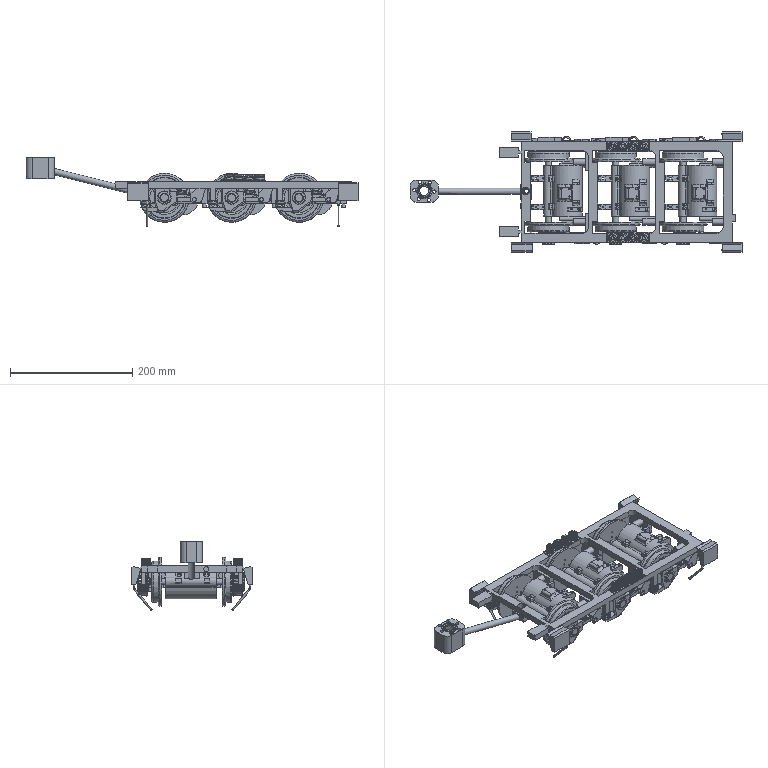Assembly | NX | mm | 34 component files | 77 solids | 1892 faces | box 542.92 x 197.4 x 112.37 mm | volume 1368528 mm3 | plane 1259 | cylinder 414 | spline 106 | sphere 64 | torus 49 | commonest cylinder face diameters 6 x108 2.235 x36 2.354 x36 7.6 x18 4.56 x12 10 x10 20 x10 10.2 x9
Bill of materials:
unnamed part 1 | 6 |  | Compact multi-body bracket/latch-like piece: blocky central body with a raised rounded-rectangle top pad and a circular boss with concentric stepped rings on one face, a curved-bottom wedge-shaped flange projecting to one side, and a slender bar extending the other way to an angled plate tab with a round through-hole.
unnamed part 2 | 1 |  | Rectangular ladder-style open frame: two long side rails joined by end and intermediate cross members, making three open bays. Small blocks and short cylindrical pins hang below, block-shaped end pieces sit at the four corners, thin angled rods extend downward and outward at the ends, and small raised studs run in a row along parts of the rails.
unnamed part 3 | 3 |  | Wheel-and-axle-like body: two identical flanged discs on the ends of a straight cylindrical shaft. Each disc has a larger-diameter flange lip on its inner side, a recessed face, and a ring pattern of small round holes or dimples. The shaft ends stick out a little past the discs.
unnamed part 4 | 3 |  | Large cylindrical body with a smaller parallel tube along one side. Raised saddle/rib features and a square mounting pad with small holes sit on top, and two flat perforated strip tabs stick out sideways. The end face has an off-center through-hole, a lug ring around the side tube bore, and a straight arm extending from that lug.
unnamed part 5 | 20 |  | Helical coil of round-section wire wound closely, about 7–8 turns, with a flat ground-style annular face at the top end and an open bore through the center.
unnamed part 6 | 1 |  | Two blocks joined by a long straight cylindrical rod: a larger rounded-square block with a central bore, an encircling ring of small spherical bumps, and four corner holes, and a small rectangular block at the far end with its own small bore ringed by small bumps. The rod meets the large block on its side face and runs at an angle.
Mates:
1. touch align | wheel_hub 3 face | frame 1 face
2. distance | lun_gu 3 face | frame 1 face
3. distance | spring 20 face | outer_hub 6 face
4. distance | outer_hub 6 face | frame 1 face
5. fix | assembly component
6. bond | 11 4 component | assembly component
7. bond | 11 3 component | assembly component
8. linear | assembly datumaxis | assembly cartesiancoordinatesystem | assembly cartesiancoordinatesystem
9. fix | assembly component
10. bond | spring 20 component | assembly component
11. bond | 11 4 component | assembly component
12. bond | spring_11 1 component | assembly component
13. bond | lun_gu 3 component | assembly component
14. bond | wheel_hub 3 component | assembly component
15. bond | outer_hub 6 component | assembly component
16. bond | 11 3 component | assembly component
17. bond | assembly component
18. bond | assembly component
19. bond | assembly component
20. bond | assembly component
21. bond | assembly component
22. bond | assembly component
23. bond | assembly component
24. linear | assembly datumaxis | assembly cartesiancoordinatesystem | assembly cartesiancoordinatesystem | assembly cartesiancoordinatesystem
25. linear | assembly datumaxis | assembly cartesiancoordinatesystem | assembly cartesiancoordinatesystem | assembly cartesiancoordinatesystem
26. linear | assembly datumaxis | assembly cartesiancoordinatesystem | assembly cartesiancoordinatesystem | assembly cartesiancoordinatesystem
27. linear | assembly datumaxis | assembly cartesiancoordinatesystem | assembly cartesiancoordinatesystem | assembly cartesiancoordinatesystem
28. linear | assembly datumaxis | assembly cartesiancoordinatesystem | assembly cartesiancoordinatesystem | assembly cartesiancoordinatesystem
29. linear | assembly datumaxis | assembly cartesiancoordinatesystem | assembly cartesiancoordinatesystem | assembly cartesiancoordinatesystem
30. linear | assembly datumaxis | assembly cartesiancoordinatesystem | assembly cartesiancoordinatesystem | assembly cartesiancoordinatesystem
31. bond | assembly component
32. bond | assembly component
33. bond | assembly component
34. bond | assembly component
35. bond | assembly component
36. bond | assembly component
37. bond | assembly component
38. distance | spring 19 face | outer_hub 6 face
39. distance | spring 19 face | outer_hub 6 face
40. distance | spring 18 face | frame 1 face
41. distance | spring 18 face | frame 1 face
42. distance | spring 18 face | frame 1 face
43. fix | assembly component
44. bond | spring 18 component | assembly component
45. bond | spring 17 component | assembly component
46. linear | assembly datumaxis | assembly cartesiancoordinatesystem | assembly cartesiancoordinatesystem | assembly cartesiancoordinatesystem | assembly cartesiancoordinatesystem
47. bond | spring 16 component | assembly component
48. bond | spring 15 component | assembly component
49. fix | assembly component
50. bond | spring 18 component | assembly component
51. bond | spring 15 component | assembly component
52. bond | spring 16 component | assembly component
53. bond | spring 17 component | assembly component
54. bond | spring 14 component | assembly component
55. bond | spring 13 component | assembly component
56. bond | spring 12 component | assembly component
57. bond | spring 11 component | assembly component
58. linear | assembly datumaxis | assembly cartesiancoordinatesystem | assembly cartesiancoordinatesystem
59. linear | assembly datumaxis | assembly cartesiancoordinatesystem | assembly cartesiancoordinatesystem
60. linear | assembly datumaxis | assembly cartesiancoordinatesystem | assembly cartesiancoordinatesystem
61. linear | assembly datumaxis | assembly cartesiancoordinatesystem | assembly cartesiancoordinatesystem
62. fix | assembly component
63. bond | spring 20 component | assembly component
64. bond | lun_gu 3 component | assembly component
65. bond | wheel_hub 3 component | assembly component
66. bond | outer_hub 6 component | assembly component
67. bond | 11 3 component | assembly component
68. bond | spring 19 component | assembly component
69. bond | spring 10 component | assembly component
70. bond | lun_gu 2 component | assembly component
71. bond | wheel_hub 2 component | assembly component
72. bond | outer_hub 5 component | assembly component
73. bond | 11 2 component | assembly component
74. bond | spring 9 component | assembly component
75. linear | assembly datumaxis | assembly cartesiancoordinatesystem | assembly cartesiancoordinatesystem | assembly cartesiancoordinatesystem
76. linear | assembly datumaxis | assembly cartesiancoordinatesystem | assembly cartesiancoordinatesystem | assembly cartesiancoordinatesystem
77. linear | assembly datumaxis | assembly cartesiancoordinatesystem | assembly cartesiancoordinatesystem | assembly cartesiancoordinatesystem
78. linear | assembly datumaxis | assembly cartesiancoordinatesystem | assembly cartesiancoordinatesystem | assembly cartesiancoordinatesystem
79. linear | assembly datumaxis | assembly cartesiancoordinatesystem | assembly cartesiancoordinatesystem | assembly cartesiancoordinatesystem
80. linear | assembly datumaxis | assembly cartesiancoordinatesystem | assembly cartesiancoordinatesystem | assembly cartesiancoordinatesystem
81. bond | spring 8 component | assembly component
82. bond | lun_gu 1 component | assembly component
83. bond | wheel_hub 1 component | assembly component
84. bond | outer_hub 4 component | assembly component
85. bond | 11 1 component | assembly component
86. bond | spring 7 component | assembly component
87. fix | assembly component
88. bond | spring 10 component | assembly component
89. bond | spring 20 component | assembly component
90. bond | outer_hub 6 component | assembly component
91. bond | spring 19 component | assembly component
92. bond | outer_hub 4 component | assembly component
93. bond | spring 7 component | assembly component
94. bond | spring 8 component | assembly component
95. bond | spring 9 component | assembly component
96. bond | outer_hub 5 component | assembly component
97. bond | spring 6 component | assembly component
98. bond | spring 5 component | assembly component
99. bond | outer_hub 3 component | assembly component
100. bond | spring 4 component | assembly component
101. bond | outer_hub 2 component | assembly component
102. bond | spring 3 component | assembly component
103. bond | spring 2 component | assembly component
104. bond | spring 1 component | assembly component
105. bond | outer_hub 1 component | assembly component
106. linear | assembly datumaxis | assembly cartesiancoordinatesystem | assembly cartesiancoordinatesystem
107. linear | assembly datumaxis | assembly cartesiancoordinatesystem | assembly cartesiancoordinatesystem
108. linear | assembly datumaxis | assembly cartesiancoordinatesystem | assembly cartesiancoordinatesystem
109. linear | assembly datumaxis | assembly cartesiancoordinatesystem | assembly cartesiancoordinatesystem
110. linear | assembly datumaxis | assembly cartesiancoordinatesystem | assembly cartesiancoordinatesystem
111. linear | assembly datumaxis | assembly cartesiancoordinatesystem | assembly cartesiancoordinatesystem
112. linear | assembly datumaxis | assembly cartesiancoordinatesystem | assembly cartesiancoordinatesystem
113. linear | assembly datumaxis | assembly cartesiancoordinatesystem | assembly cartesiancoordinatesystem
114. linear | assembly datumaxis | assembly cartesiancoordinatesystem | assembly cartesiancoordinatesystem
115. distance | red 1 face | frame 1 face
116. distance | red 1 face | frame 1 face
117. distance | red 1 face | frame 1 face
118. align lock | outer_hub 6 face | wheel_hub 3 face